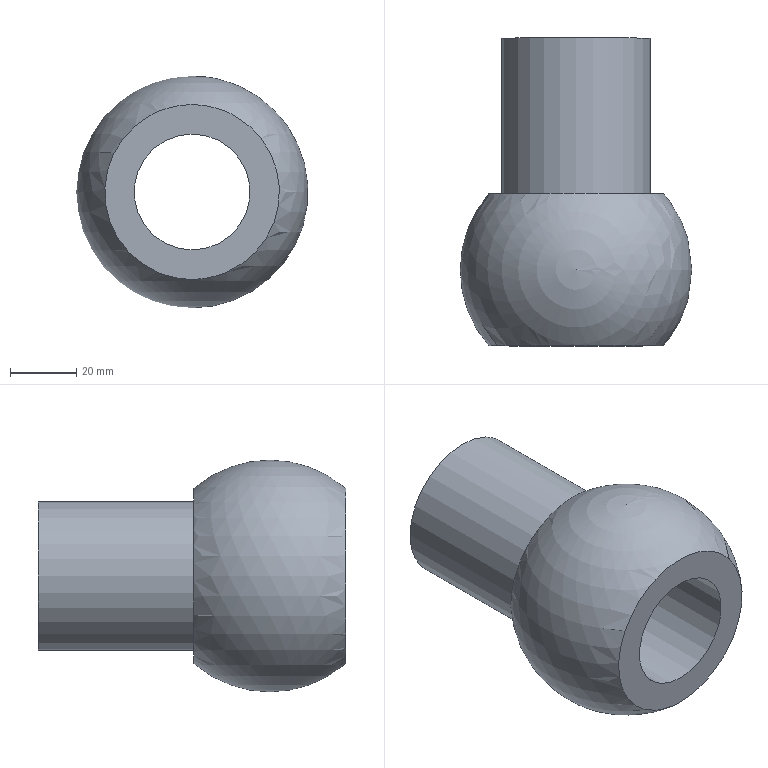Component | NX | BALL_JOINT | 1 solid | 6 faces | box 70 x 105 x 70 mm | volume 136818 mm3 | plane 3 | cylinder 2 | sphere 1 | commonest cylinder face diameters 45 x1 35 x1
STEP:
#1=CARTESIAN_POINT('',(0.,0.,0.));
#2=DIRECTION('',(0.,0.,1.));
#3=DIRECTION('',(1.,0.,0.));
#4=AXIS2_PLACEMENT_3D('',#1,#2,#3);
#5=CARTESIAN_POINT('',(183.939,23.,87.004));
#6=VERTEX_POINT('',#5);
#7=CARTESIAN_POINT('',(183.939,23.,60.622));
#8=DIRECTION('',(0.,-1.,0.));
#9=DIRECTION('',(0.,0.,1.));
#10=AXIS2_PLACEMENT_3D('',#7,#8,#9);
#11=CIRCLE('',#10,26.382);
#12=CARTESIAN_POINT('',(183.939,-0.,60.622));
#13=DIRECTION('',(0.,0.,1.));
#14=DIRECTION('',(1.,0.,0.));
#15=AXIS2_PLACEMENT_3D('',#12,#13,#14);
#16=SPHERICAL_SURFACE('',#15,35.);
#17=CARTESIAN_POINT('',(7.854,0.8538));
#18=CARTESIAN_POINT('',(7.968,0.8544));
#19=CARTESIAN_POINT('',(8.178,0.8212));
#20=CARTESIAN_POINT('',(8.424,0.6948));
#21=CARTESIAN_POINT('',(8.579,0.5205));
#22=CARTESIAN_POINT('',(8.669,0.3206));
#23=CARTESIAN_POINT('',(8.709,0.1081));
#24=CARTESIAN_POINT('',(8.709,-0.1081));
#25=CARTESIAN_POINT('',(8.669,-0.3206));
#26=CARTESIAN_POINT('',(8.579,-0.5205));
#27=CARTESIAN_POINT('',(8.424,-0.6948));
#28=CARTESIAN_POINT('',(8.18,-0.8215));
#29=CARTESIAN_POINT('',(7.854,-0.8699));
#30=CARTESIAN_POINT('',(7.528,-0.8215));
#31=CARTESIAN_POINT('',(7.284,-0.6948));
#32=CARTESIAN_POINT('',(7.129,-0.5205));
#33=CARTESIAN_POINT('',(7.039,-0.3206));
#34=CARTESIAN_POINT('',(6.998,-0.1081));
#35=CARTESIAN_POINT('',(6.999,0.1081));
#36=CARTESIAN_POINT('',(7.039,0.3206));
#37=CARTESIAN_POINT('',(7.129,0.5205));
#38=CARTESIAN_POINT('',(7.284,0.6948));
#39=CARTESIAN_POINT('',(7.53,0.8212));
#40=CARTESIAN_POINT('',(7.74,0.8544));
#41=CARTESIAN_POINT('',(7.854,0.8538));
#42=B_SPLINE_CURVE_WITH_KNOTS('',3,(#17,#18,#19,#20,#21,#22,#23,#24,#25,#26,#27,#28,#29,#30,#31,#32,#33,#34,#35,#36,#37,#38,#39,#40,#41),.UNSPECIFIED.,.T.,.F.,(4,1,1,1,1,1,1,1,1,1,1,1,1,1,1,1,1,1,1,1,1,1,4),(0.,0.2856,0.5712,0.8568,1.142,1.428,1.714,1.999,2.285,2.57,2.856,3.142,3.427,3.713,3.998,4.284,4.57,4.855,5.141,5.426,5.712,5.998,6.283),.QUASI_UNIFORM_KNOTS.);
#43=(GEOMETRIC_REPRESENTATION_CONTEXT(2)PARAMETRIC_REPRESENTATION_CONTEXT()REPRESENTATION_CONTEXT('',''));
#44=DEFINITIONAL_REPRESENTATION('',(#42),#43);
#45=PCURVE('',#16,#44);
#46=CARTESIAN_POINT('',(183.939,23.,60.622));
#47=DIRECTION('',(0.,1.,0.));
#48=DIRECTION('',(0.,0.,1.));
#49=AXIS2_PLACEMENT_3D('',#46,#47,#48);
#50=PLANE('',#49);
#51=CARTESIAN_POINT('',(26.382,0.));
#52=CARTESIAN_POINT('',(26.382,-45.695));
#53=CARTESIAN_POINT('',(-13.191,-22.847));
#54=CARTESIAN_POINT('',(-52.764,-0.));
#55=CARTESIAN_POINT('',(-13.191,22.847));
#56=CARTESIAN_POINT('',(26.382,45.695));
#57=CARTESIAN_POINT('',(26.382,0.));
#58=(BOUNDED_CURVE()B_SPLINE_CURVE(2,(#51,#52,#53,#54,#55,#56,#57),.UNSPECIFIED.,.T.,.F.)B_SPLINE_CURVE_WITH_KNOTS((1,2,2,2,2,1),(-2.094,0.,2.094,4.189,6.283,8.378),.UNSPECIFIED.)CURVE()GEOMETRIC_REPRESENTATION_ITEM()RATIONAL_B_SPLINE_CURVE((1.,0.5,1.,0.5,1.,0.5,1.))REPRESENTATION_ITEM(''));
#59=(GEOMETRIC_REPRESENTATION_CONTEXT(2)PARAMETRIC_REPRESENTATION_CONTEXT()REPRESENTATION_CONTEXT('',''));
#60=DEFINITIONAL_REPRESENTATION('',(#58),#59);
#61=PCURVE('',#50,#60);
#62=SURFACE_CURVE('',#11,(#45,#61),.PCURVE_S1.);
#63=EDGE_CURVE('',#6,#6,#62,.T.);
#64=ORIENTED_EDGE('',*,*,#63,.T.);
#65=EDGE_LOOP('',(#64));
#66=FACE_BOUND('',#65,.T.);
#67=CARTESIAN_POINT('',(183.939,-23.,34.24));
#68=VERTEX_POINT('',#67);
#69=CARTESIAN_POINT('',(183.939,-23.,60.622));
#70=DIRECTION('',(0.,1.,0.));
#71=DIRECTION('',(0.,0.,-1.));
#72=AXIS2_PLACEMENT_3D('',#69,#70,#71);
#73=CIRCLE('',#72,26.382);
#74=CARTESIAN_POINT('',(4.712,-0.8538));
#75=CARTESIAN_POINT('',(4.598,-0.8544));
#76=CARTESIAN_POINT('',(4.389,-0.8212));
#77=CARTESIAN_POINT('',(4.142,-0.6948));
#78=CARTESIAN_POINT('',(3.987,-0.5205));
#79=CARTESIAN_POINT('',(3.898,-0.3206));
#80=CARTESIAN_POINT('',(3.857,-0.1081));
#81=CARTESIAN_POINT('',(3.857,0.1081));
#82=CARTESIAN_POINT('',(3.898,0.3206));
#83=CARTESIAN_POINT('',(3.987,0.5205));
#84=CARTESIAN_POINT('',(4.143,0.6948));
#85=CARTESIAN_POINT('',(4.386,0.8215));
#86=CARTESIAN_POINT('',(4.712,0.8699));
#87=CARTESIAN_POINT('',(5.039,0.8215));
#88=CARTESIAN_POINT('',(5.282,0.6948));
#89=CARTESIAN_POINT('',(5.438,0.5205));
#90=CARTESIAN_POINT('',(5.527,0.3206));
#91=CARTESIAN_POINT('',(5.568,0.1081));
#92=CARTESIAN_POINT('',(5.568,-0.1081));
#93=CARTESIAN_POINT('',(5.527,-0.3206));
#94=CARTESIAN_POINT('',(5.437,-0.5205));
#95=CARTESIAN_POINT('',(5.283,-0.6948));
#96=CARTESIAN_POINT('',(5.036,-0.8212));
#97=CARTESIAN_POINT('',(4.827,-0.8544));
#98=CARTESIAN_POINT('',(4.712,-0.8538));
#99=B_SPLINE_CURVE_WITH_KNOTS('',3,(#74,#75,#76,#77,#78,#79,#80,#81,#82,#83,#84,#85,#86,#87,#88,#89,#90,#91,#92,#93,#94,#95,#96,#97,#98),.UNSPECIFIED.,.T.,.F.,(4,1,1,1,1,1,1,1,1,1,1,1,1,1,1,1,1,1,1,1,1,1,4),(0.,0.2856,0.5712,0.8568,1.142,1.428,1.714,1.999,2.285,2.57,2.856,3.142,3.427,3.713,3.998,4.284,4.57,4.855,5.141,5.426,5.712,5.998,6.283),.QUASI_UNIFORM_KNOTS.);
#100=(GEOMETRIC_REPRESENTATION_CONTEXT(2)PARAMETRIC_REPRESENTATION_CONTEXT()REPRESENTATION_CONTEXT('',''));
#101=DEFINITIONAL_REPRESENTATION('',(#99),#100);
#102=PCURVE('',#16,#101);
#103=CARTESIAN_POINT('',(183.939,-23.,60.622));
#104=DIRECTION('',(0.,-1.,0.));
#105=DIRECTION('',(0.,0.,-1.));
#106=AXIS2_PLACEMENT_3D('',#103,#104,#105);
#107=PLANE('',#106);
#108=CARTESIAN_POINT('',(26.382,0.));
#109=CARTESIAN_POINT('',(26.382,-45.695));
#110=CARTESIAN_POINT('',(-13.191,-22.847));
#111=CARTESIAN_POINT('',(-52.764,-0.));
#112=CARTESIAN_POINT('',(-13.191,22.847));
#113=CARTESIAN_POINT('',(26.382,45.695));
#114=CARTESIAN_POINT('',(26.382,0.));
#115=(BOUNDED_CURVE()B_SPLINE_CURVE(2,(#108,#109,#110,#111,#112,#113,#114),.UNSPECIFIED.,.T.,.F.)B_SPLINE_CURVE_WITH_KNOTS((1,2,2,2,2,1),(-2.094,0.,2.094,4.189,6.283,8.378),.UNSPECIFIED.)CURVE()GEOMETRIC_REPRESENTATION_ITEM()RATIONAL_B_SPLINE_CURVE((1.,0.5,1.,0.5,1.,0.5,1.))REPRESENTATION_ITEM(''));
#116=(GEOMETRIC_REPRESENTATION_CONTEXT(2)PARAMETRIC_REPRESENTATION_CONTEXT()REPRESENTATION_CONTEXT('',''));
#117=DEFINITIONAL_REPRESENTATION('',(#115),#116);
#118=PCURVE('',#107,#117);
#119=SURFACE_CURVE('',#73,(#102,#118),.PCURVE_S1.);
#120=EDGE_CURVE('',#68,#68,#119,.T.);
#121=ORIENTED_EDGE('',*,*,#120,.T.);
#122=EDGE_LOOP('',(#121));
#123=FACE_BOUND('',#122,.T.);
#124=CARTESIAN_POINT('',(183.939,-0.,25.622));
#125=VERTEX_POINT('',#124);
#126=VERTEX_LOOP('',#125);
#127=FACE_BOUND('',#126,.T.);
#128=ADVANCED_FACE('',(#66,#123,#127),#16,.T.);
#129=CARTESIAN_POINT('',(183.939,23.,83.122));
#130=VERTEX_POINT('',#129);
#131=CARTESIAN_POINT('',(206.439,23.,60.622));
#132=VERTEX_POINT('',#131);
#133=CARTESIAN_POINT('',(183.939,23.,60.622));
#134=DIRECTION('',(0.,1.,0.));
#135=DIRECTION('',(0.,0.,1.));
#136=AXIS2_PLACEMENT_3D('',#133,#134,#135);
#137=CIRCLE('',#136,22.5);
#138=CARTESIAN_POINT('',(0.,0.));
#139=DIRECTION('',(1.,0.));
#140=AXIS2_PLACEMENT_2D('',#138,#139);
#141=CIRCLE('',#140,22.5);
#142=(GEOMETRIC_REPRESENTATION_CONTEXT(2)PARAMETRIC_REPRESENTATION_CONTEXT()REPRESENTATION_CONTEXT('',''));
#143=DEFINITIONAL_REPRESENTATION('',(#141),#142);
#144=PCURVE('',#50,#143);
#145=CARTESIAN_POINT('',(183.939,70.,60.622));
#146=DIRECTION('',(0.,-1.,0.));
#147=DIRECTION('',(0.,0.,-1.));
#148=AXIS2_PLACEMENT_3D('',#145,#146,#147);
#149=CYLINDRICAL_SURFACE('',#148,22.5);
#150=CARTESIAN_POINT('',(3.142,47.));
#151=DIRECTION('',(-1.,0.));
#152=VECTOR('',#151,1.);
#153=LINE('',#150,#152);
#154=(GEOMETRIC_REPRESENTATION_CONTEXT(2)PARAMETRIC_REPRESENTATION_CONTEXT()REPRESENTATION_CONTEXT('',''));
#155=DEFINITIONAL_REPRESENTATION('',(#153),#154);
#156=PCURVE('',#149,#155);
#157=SURFACE_CURVE('',#137,(#144,#156),.PCURVE_S1.);
#158=EDGE_CURVE('',#130,#132,#157,.T.);
#159=ORIENTED_EDGE('',*,*,#158,.F.);
#160=CARTESIAN_POINT('',(183.939,23.,60.622));
#161=DIRECTION('',(0.,1.,0.));
#162=DIRECTION('',(0.,0.,1.));
#163=AXIS2_PLACEMENT_3D('',#160,#161,#162);
#164=CIRCLE('',#163,22.5);
#165=CARTESIAN_POINT('',(0.,0.));
#166=DIRECTION('',(1.,0.));
#167=AXIS2_PLACEMENT_2D('',#165,#166);
#168=CIRCLE('',#167,22.5);
#169=(GEOMETRIC_REPRESENTATION_CONTEXT(2)PARAMETRIC_REPRESENTATION_CONTEXT()REPRESENTATION_CONTEXT('',''));
#170=DEFINITIONAL_REPRESENTATION('',(#168),#169);
#171=PCURVE('',#50,#170);
#172=CARTESIAN_POINT('',(9.425,47.));
#173=DIRECTION('',(-1.,0.));
#174=VECTOR('',#173,1.);
#175=LINE('',#172,#174);
#176=(GEOMETRIC_REPRESENTATION_CONTEXT(2)PARAMETRIC_REPRESENTATION_CONTEXT()REPRESENTATION_CONTEXT('',''));
#177=DEFINITIONAL_REPRESENTATION('',(#175),#176);
#178=PCURVE('',#149,#177);
#179=SURFACE_CURVE('',#164,(#171,#178),.PCURVE_S1.);
#180=EDGE_CURVE('',#132,#130,#179,.T.);
#181=ORIENTED_EDGE('',*,*,#180,.F.);
#182=EDGE_LOOP('',(#159,#181));
#183=FACE_BOUND('',#182,.T.);
#184=ORIENTED_EDGE('',*,*,#63,.F.);
#185=EDGE_LOOP('',(#184));
#186=FACE_BOUND('',#185,.T.);
#187=ADVANCED_FACE('',(#183,#186),#50,.T.);
#188=CARTESIAN_POINT('',(183.939,-23.,78.122));
#189=VERTEX_POINT('',#188);
#190=CARTESIAN_POINT('',(183.939,-23.,60.622));
#191=DIRECTION('',(0.,1.,0.));
#192=DIRECTION('',(0.,0.,1.));
#193=AXIS2_PLACEMENT_3D('',#190,#191,#192);
#194=CIRCLE('',#193,17.5);
#195=CARTESIAN_POINT('',(-17.5,0.));
#196=CARTESIAN_POINT('',(-17.5,30.311));
#197=CARTESIAN_POINT('',(8.75,15.155));
#198=CARTESIAN_POINT('',(35.,0.));
#199=CARTESIAN_POINT('',(8.75,-15.155));
#200=CARTESIAN_POINT('',(-17.5,-30.311));
#201=CARTESIAN_POINT('',(-17.5,0.));
#202=(BOUNDED_CURVE()B_SPLINE_CURVE(2,(#195,#196,#197,#198,#199,#200,#201),.UNSPECIFIED.,.T.,.F.)B_SPLINE_CURVE_WITH_KNOTS((1,2,2,2,2,1),(-2.094,0.,2.094,4.189,6.283,8.378),.UNSPECIFIED.)CURVE()GEOMETRIC_REPRESENTATION_ITEM()RATIONAL_B_SPLINE_CURVE((1.,0.5,1.,0.5,1.,0.5,1.))REPRESENTATION_ITEM(''));
#203=(GEOMETRIC_REPRESENTATION_CONTEXT(2)PARAMETRIC_REPRESENTATION_CONTEXT()REPRESENTATION_CONTEXT('',''));
#204=DEFINITIONAL_REPRESENTATION('',(#202),#203);
#205=PCURVE('',#107,#204);
#206=CARTESIAN_POINT('',(183.939,-23.,60.622));
#207=DIRECTION('',(0.,1.,0.));
#208=DIRECTION('',(0.,0.,1.));
#209=AXIS2_PLACEMENT_3D('',#206,#207,#208);
#210=CYLINDRICAL_SURFACE('',#209,17.5);
#211=CARTESIAN_POINT('',(0.,0.));
#212=DIRECTION('',(1.,0.));
#213=VECTOR('',#212,1.);
#214=LINE('',#211,#213);
#215=(GEOMETRIC_REPRESENTATION_CONTEXT(2)PARAMETRIC_REPRESENTATION_CONTEXT()REPRESENTATION_CONTEXT('',''));
#216=DEFINITIONAL_REPRESENTATION('',(#214),#215);
#217=PCURVE('',#210,#216);
#218=SURFACE_CURVE('',#194,(#205,#217),.PCURVE_S1.);
#219=EDGE_CURVE('',#189,#189,#218,.T.);
#220=ORIENTED_EDGE('',*,*,#219,.T.);
#221=EDGE_LOOP('',(#220));
#222=FACE_BOUND('',#221,.T.);
#223=ORIENTED_EDGE('',*,*,#120,.F.);
#224=EDGE_LOOP('',(#223));
#225=FACE_BOUND('',#224,.T.);
#226=ADVANCED_FACE('',(#222,#225),#107,.T.);
#227=ORIENTED_EDGE('',*,*,#158,.T.);
#228=CARTESIAN_POINT('',(206.439,70.,60.622));
#229=VERTEX_POINT('',#228);
#230=CARTESIAN_POINT('',(206.439,70.,60.622));
#231=CARTESIAN_POINT('',(206.439,23.,60.622));
#232=B_SPLINE_CURVE_WITH_KNOTS('',1,(#230,#231),.UNSPECIFIED.,.F.,.F.,(2,2),(0.,47.),.PIECEWISE_BEZIER_KNOTS.);
#233=CARTESIAN_POINT('',(1.571,0.));
#234=DIRECTION('',(0.,1.));
#235=VECTOR('',#234,1.);
#236=LINE('',#233,#235);
#237=(GEOMETRIC_REPRESENTATION_CONTEXT(2)PARAMETRIC_REPRESENTATION_CONTEXT()REPRESENTATION_CONTEXT('',''));
#238=DEFINITIONAL_REPRESENTATION('',(#236),#237);
#239=PCURVE('',#149,#238);
#240=CARTESIAN_POINT('',(7.854,0.));
#241=DIRECTION('',(0.,1.));
#242=VECTOR('',#241,1.);
#243=LINE('',#240,#242);
#244=(GEOMETRIC_REPRESENTATION_CONTEXT(2)PARAMETRIC_REPRESENTATION_CONTEXT()REPRESENTATION_CONTEXT('',''));
#245=DEFINITIONAL_REPRESENTATION('',(#243),#244);
#246=PCURVE('',#149,#245);
#247=SEAM_CURVE('',#232,(#239,#246),.PCURVE_S1.);
#248=EDGE_CURVE('',#229,#132,#247,.T.);
#249=ORIENTED_EDGE('',*,*,#248,.F.);
#250=CARTESIAN_POINT('',(183.939,70.,60.622));
#251=DIRECTION('',(0.,-1.,0.));
#252=DIRECTION('',(1.,0.,0.));
#253=AXIS2_PLACEMENT_3D('',#250,#251,#252);
#254=CIRCLE('',#253,22.5);
#255=CARTESIAN_POINT('',(1.571,0.));
#256=DIRECTION('',(1.,0.));
#257=VECTOR('',#256,1.);
#258=LINE('',#255,#257);
#259=(GEOMETRIC_REPRESENTATION_CONTEXT(2)PARAMETRIC_REPRESENTATION_CONTEXT()REPRESENTATION_CONTEXT('',''));
#260=DEFINITIONAL_REPRESENTATION('',(#258),#259);
#261=PCURVE('',#149,#260);
#262=CARTESIAN_POINT('',(183.939,70.,60.622));
#263=DIRECTION('',(0.,1.,0.));
#264=DIRECTION('',(0.,0.,1.));
#265=AXIS2_PLACEMENT_3D('',#262,#263,#264);
#266=PLANE('',#265);
#267=CARTESIAN_POINT('',(0.,22.5));
#268=CARTESIAN_POINT('',(38.971,22.5));
#269=CARTESIAN_POINT('',(19.486,-11.25));
#270=CARTESIAN_POINT('',(0.,-45.));
#271=CARTESIAN_POINT('',(-19.486,-11.25));
#272=CARTESIAN_POINT('',(-38.971,22.5));
#273=CARTESIAN_POINT('',(0.,22.5));
#274=(BOUNDED_CURVE()B_SPLINE_CURVE(2,(#267,#268,#269,#270,#271,#272,#273),.UNSPECIFIED.,.T.,.F.)B_SPLINE_CURVE_WITH_KNOTS((1,2,2,2,2,1),(-2.094,0.,2.094,4.189,6.283,8.378),.UNSPECIFIED.)CURVE()GEOMETRIC_REPRESENTATION_ITEM()RATIONAL_B_SPLINE_CURVE((1.,0.5,1.,0.5,1.,0.5,1.))REPRESENTATION_ITEM(''));
#275=(GEOMETRIC_REPRESENTATION_CONTEXT(2)PARAMETRIC_REPRESENTATION_CONTEXT()REPRESENTATION_CONTEXT('',''));
#276=DEFINITIONAL_REPRESENTATION('',(#274),#275);
#277=PCURVE('',#266,#276);
#278=SURFACE_CURVE('',#254,(#261,#277),.PCURVE_S1.);
#279=EDGE_CURVE('',#229,#229,#278,.T.);
#280=ORIENTED_EDGE('',*,*,#279,.T.);
#281=ORIENTED_EDGE('',*,*,#248,.T.);
#282=ORIENTED_EDGE('',*,*,#180,.T.);
#283=EDGE_LOOP('',(#227,#249,#280,#281,#282));
#284=FACE_BOUND('',#283,.T.);
#285=ADVANCED_FACE('',(#284),#149,.T.);
#286=CARTESIAN_POINT('',(183.939,70.,78.122));
#287=VERTEX_POINT('',#286);
#288=CARTESIAN_POINT('',(183.939,70.,60.622));
#289=DIRECTION('',(0.,1.,0.));
#290=DIRECTION('',(0.,0.,1.));
#291=AXIS2_PLACEMENT_3D('',#288,#289,#290);
#292=CIRCLE('',#291,17.5);
#293=CARTESIAN_POINT('',(0.,0.));
#294=DIRECTION('',(1.,0.));
#295=AXIS2_PLACEMENT_2D('',#293,#294);
#296=CIRCLE('',#295,17.5);
#297=(GEOMETRIC_REPRESENTATION_CONTEXT(2)PARAMETRIC_REPRESENTATION_CONTEXT()REPRESENTATION_CONTEXT('',''));
#298=DEFINITIONAL_REPRESENTATION('',(#296),#297);
#299=PCURVE('',#266,#298);
#300=CARTESIAN_POINT('',(0.,93.));
#301=DIRECTION('',(1.,0.));
#302=VECTOR('',#301,1.);
#303=LINE('',#300,#302);
#304=(GEOMETRIC_REPRESENTATION_CONTEXT(2)PARAMETRIC_REPRESENTATION_CONTEXT()REPRESENTATION_CONTEXT('',''));
#305=DEFINITIONAL_REPRESENTATION('',(#303),#304);
#306=PCURVE('',#210,#305);
#307=SURFACE_CURVE('',#292,(#299,#306),.PCURVE_S1.);
#308=EDGE_CURVE('',#287,#287,#307,.T.);
#309=ORIENTED_EDGE('',*,*,#308,.F.);
#310=EDGE_LOOP('',(#309));
#311=FACE_BOUND('',#310,.T.);
#312=ORIENTED_EDGE('',*,*,#279,.F.);
#313=EDGE_LOOP('',(#312));
#314=FACE_BOUND('',#313,.T.);
#315=ADVANCED_FACE('',(#311,#314),#266,.T.);
#316=ORIENTED_EDGE('',*,*,#308,.F.);
#317=CARTESIAN_POINT('',(183.939,-23.,78.122));
#318=CARTESIAN_POINT('',(183.939,70.,78.122));
#319=B_SPLINE_CURVE_WITH_KNOTS('',1,(#317,#318),.UNSPECIFIED.,.F.,.F.,(2,2),(0.,93.),.PIECEWISE_BEZIER_KNOTS.);
#320=CARTESIAN_POINT('',(0.,0.));
#321=DIRECTION('',(0.,1.));
#322=VECTOR('',#321,1.);
#323=LINE('',#320,#322);
#324=(GEOMETRIC_REPRESENTATION_CONTEXT(2)PARAMETRIC_REPRESENTATION_CONTEXT()REPRESENTATION_CONTEXT('',''));
#325=DEFINITIONAL_REPRESENTATION('',(#323),#324);
#326=PCURVE('',#210,#325);
#327=CARTESIAN_POINT('',(6.283,0.));
#328=DIRECTION('',(0.,1.));
#329=VECTOR('',#328,1.);
#330=LINE('',#327,#329);
#331=(GEOMETRIC_REPRESENTATION_CONTEXT(2)PARAMETRIC_REPRESENTATION_CONTEXT()REPRESENTATION_CONTEXT('',''));
#332=DEFINITIONAL_REPRESENTATION('',(#330),#331);
#333=PCURVE('',#210,#332);
#334=SEAM_CURVE('',#319,(#326,#333),.PCURVE_S1.);
#335=EDGE_CURVE('',#189,#287,#334,.T.);
#336=ORIENTED_EDGE('',*,*,#335,.F.);
#337=ORIENTED_EDGE('',*,*,#219,.T.);
#338=ORIENTED_EDGE('',*,*,#335,.T.);
#339=EDGE_LOOP('',(#316,#336,#337,#338));
#340=FACE_BOUND('',#339,.F.);
#341=ADVANCED_FACE('',(#340),#210,.F.);
#342=CLOSED_SHELL('',(#128,#187,#226,#285,#315,#341));
#343=MANIFOLD_SOLID_BREP('',#342);
#344=(LENGTH_UNIT()NAMED_UNIT(*)SI_UNIT(.MILLI.,.METRE.));
#345=UNCERTAINTY_MEASURE_WITH_UNIT(LENGTH_MEASURE(0.000005),#344,'','');
#346=(NAMED_UNIT(*)PLANE_ANGLE_UNIT()SI_UNIT($,.RADIAN.));
#347=(NAMED_UNIT(*)SI_UNIT($,.STERADIAN.)SOLID_ANGLE_UNIT());
#348=(GEOMETRIC_REPRESENTATION_CONTEXT(3)GLOBAL_UNCERTAINTY_ASSIGNED_CONTEXT((#345))GLOBAL_UNIT_ASSIGNED_CONTEXT((#344,#346,#347))REPRESENTATION_CONTEXT('',''));
#349=ADVANCED_BREP_SHAPE_REPRESENTATION('',(#4,#343),#348);